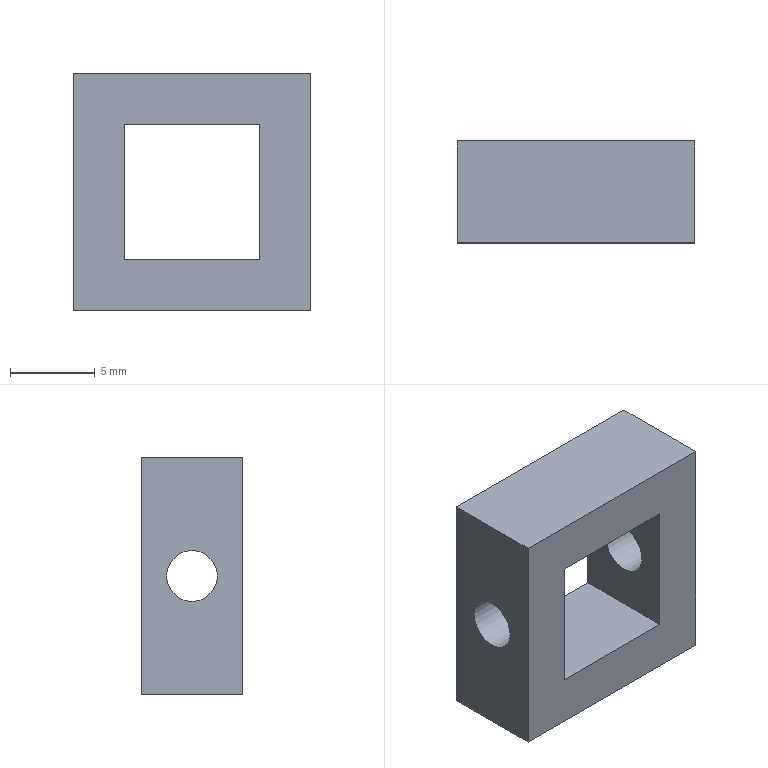Component | NX | PISTON_BLOCK_ASSEMBLY | 1 solid | 12 faces | box 14 x 6 x 14 mm | volume 750 mm3 | plane 10 | cylinder 2 | commonest cylinder face diameters 3 x2
STEP:
#1=CARTESIAN_POINT('',(0.,0.,0.));
#2=DIRECTION('',(0.,0.,1.));
#3=DIRECTION('',(1.,0.,0.));
#4=AXIS2_PLACEMENT_3D('',#1,#2,#3);
#5=CARTESIAN_POINT('',(-96.724,-9.25,41.));
#6=VERTEX_POINT('',#5);
#7=CARTESIAN_POINT('',(-96.724,-10.75,41.));
#8=DIRECTION('',(-1.,0.,0.));
#9=DIRECTION('',(0.,1.,0.));
#10=AXIS2_PLACEMENT_3D('',#7,#8,#9);
#11=CIRCLE('',#10,1.5);
#12=CARTESIAN_POINT('',(-96.724,-7.75,45.));
#13=DIRECTION('',(-1.,0.,0.));
#14=DIRECTION('',(0.,1.,0.));
#15=AXIS2_PLACEMENT_3D('',#12,#13,#14);
#16=PLANE('',#15);
#17=CARTESIAN_POINT('',(-3.,4.));
#18=DIRECTION('',(1.,0.));
#19=AXIS2_PLACEMENT_2D('',#17,#18);
#20=CIRCLE('',#19,1.5);
#21=(GEOMETRIC_REPRESENTATION_CONTEXT(2)PARAMETRIC_REPRESENTATION_CONTEXT()REPRESENTATION_CONTEXT('',''));
#22=DEFINITIONAL_REPRESENTATION('',(#20),#21);
#23=PCURVE('',#16,#22);
#24=CARTESIAN_POINT('',(-85.724,-10.75,41.));
#25=DIRECTION('',(-1.,0.,0.));
#26=DIRECTION('',(0.,1.,0.));
#27=AXIS2_PLACEMENT_3D('',#24,#25,#26);
#28=CYLINDRICAL_SURFACE('',#27,1.5);
#29=CARTESIAN_POINT('',(0.,11.));
#30=DIRECTION('',(1.,0.));
#31=VECTOR('',#30,1.);
#32=LINE('',#29,#31);
#33=(GEOMETRIC_REPRESENTATION_CONTEXT(2)PARAMETRIC_REPRESENTATION_CONTEXT()REPRESENTATION_CONTEXT('',''));
#34=DEFINITIONAL_REPRESENTATION('',(#32),#33);
#35=PCURVE('',#28,#34);
#36=SURFACE_CURVE('',#11,(#23,#35),.PCURVE_S1.);
#37=EDGE_CURVE('',#6,#6,#36,.T.);
#38=ORIENTED_EDGE('',*,*,#37,.T.);
#39=EDGE_LOOP('',(#38));
#40=FACE_BOUND('',#39,.T.);
#41=CARTESIAN_POINT('',(-96.724,-13.75,45.));
#42=VERTEX_POINT('',#41);
#43=CARTESIAN_POINT('',(-96.724,-13.75,37.));
#44=VERTEX_POINT('',#43);
#45=CARTESIAN_POINT('',(-96.724,-13.75,45.));
#46=DIRECTION('',(0.,0.,-1.));
#47=VECTOR('',#46,1.);
#48=LINE('',#45,#47);
#49=CARTESIAN_POINT('',(-6.,0.));
#50=DIRECTION('',(0.,1.));
#51=VECTOR('',#50,1.);
#52=LINE('',#49,#51);
#53=(GEOMETRIC_REPRESENTATION_CONTEXT(2)PARAMETRIC_REPRESENTATION_CONTEXT()REPRESENTATION_CONTEXT('',''));
#54=DEFINITIONAL_REPRESENTATION('',(#52),#53);
#55=PCURVE('',#16,#54);
#56=CARTESIAN_POINT('',(-92.724,-13.75,41.));
#57=DIRECTION('',(0.,-1.,0.));
#58=DIRECTION('',(-1.,0.,0.));
#59=AXIS2_PLACEMENT_3D('',#56,#57,#58);
#60=PLANE('',#59);
#61=CARTESIAN_POINT('',(4.,-4.));
#62=DIRECTION('',(0.,1.));
#63=VECTOR('',#62,1.);
#64=LINE('',#61,#63);
#65=(GEOMETRIC_REPRESENTATION_CONTEXT(2)PARAMETRIC_REPRESENTATION_CONTEXT()REPRESENTATION_CONTEXT('',''));
#66=DEFINITIONAL_REPRESENTATION('',(#64),#65);
#67=PCURVE('',#60,#66);
#68=SURFACE_CURVE('',#48,(#55,#67),.PCURVE_S1.);
#69=EDGE_CURVE('',#42,#44,#68,.T.);
#70=ORIENTED_EDGE('',*,*,#69,.T.);
#71=CARTESIAN_POINT('',(-96.724,-7.75,37.));
#72=VERTEX_POINT('',#71);
#73=CARTESIAN_POINT('',(-96.724,-7.75,37.));
#74=DIRECTION('',(0.,-1.,0.));
#75=VECTOR('',#74,1.);
#76=LINE('',#73,#75);
#77=CARTESIAN_POINT('',(0.,8.));
#78=DIRECTION('',(-1.,0.));
#79=VECTOR('',#78,1.);
#80=LINE('',#77,#79);
#81=(GEOMETRIC_REPRESENTATION_CONTEXT(2)PARAMETRIC_REPRESENTATION_CONTEXT()REPRESENTATION_CONTEXT('',''));
#82=DEFINITIONAL_REPRESENTATION('',(#80),#81);
#83=PCURVE('',#16,#82);
#84=CARTESIAN_POINT('',(-96.724,-7.75,37.));
#85=DIRECTION('',(0.,0.,-1.));
#86=DIRECTION('',(0.,1.,0.));
#87=AXIS2_PLACEMENT_3D('',#84,#85,#86);
#88=PLANE('',#87);
#89=CARTESIAN_POINT('',(0.,0.));
#90=DIRECTION('',(-1.,0.));
#91=VECTOR('',#90,1.);
#92=LINE('',#89,#91);
#93=(GEOMETRIC_REPRESENTATION_CONTEXT(2)PARAMETRIC_REPRESENTATION_CONTEXT()REPRESENTATION_CONTEXT('',''));
#94=DEFINITIONAL_REPRESENTATION('',(#92),#93);
#95=PCURVE('',#88,#94);
#96=SURFACE_CURVE('',#76,(#83,#95),.PCURVE_S1.);
#97=EDGE_CURVE('',#72,#44,#96,.T.);
#98=ORIENTED_EDGE('',*,*,#97,.F.);
#99=CARTESIAN_POINT('',(-96.724,-7.75,45.));
#100=VERTEX_POINT('',#99);
#101=CARTESIAN_POINT('',(-96.724,-7.75,45.));
#102=DIRECTION('',(0.,0.,-1.));
#103=VECTOR('',#102,1.);
#104=LINE('',#101,#103);
#105=CARTESIAN_POINT('',(0.,0.));
#106=DIRECTION('',(0.,1.));
#107=VECTOR('',#106,1.);
#108=LINE('',#105,#107);
#109=(GEOMETRIC_REPRESENTATION_CONTEXT(2)PARAMETRIC_REPRESENTATION_CONTEXT()REPRESENTATION_CONTEXT('',''));
#110=DEFINITIONAL_REPRESENTATION('',(#108),#109);
#111=PCURVE('',#16,#110);
#112=CARTESIAN_POINT('',(-92.724,-7.75,41.));
#113=DIRECTION('',(0.,-1.,0.));
#114=DIRECTION('',(-1.,0.,0.));
#115=AXIS2_PLACEMENT_3D('',#112,#113,#114);
#116=PLANE('',#115);
#117=CARTESIAN_POINT('',(4.,-4.));
#118=DIRECTION('',(0.,1.));
#119=VECTOR('',#118,1.);
#120=LINE('',#117,#119);
#121=(GEOMETRIC_REPRESENTATION_CONTEXT(2)PARAMETRIC_REPRESENTATION_CONTEXT()REPRESENTATION_CONTEXT('',''));
#122=DEFINITIONAL_REPRESENTATION('',(#120),#121);
#123=PCURVE('',#116,#122);
#124=SURFACE_CURVE('',#104,(#111,#123),.PCURVE_S1.);
#125=EDGE_CURVE('',#100,#72,#124,.T.);
#126=ORIENTED_EDGE('',*,*,#125,.F.);
#127=CARTESIAN_POINT('',(-96.724,-7.75,45.));
#128=DIRECTION('',(0.,-1.,0.));
#129=VECTOR('',#128,1.);
#130=LINE('',#127,#129);
#131=CARTESIAN_POINT('',(0.,0.));
#132=DIRECTION('',(-1.,0.));
#133=VECTOR('',#132,1.);
#134=LINE('',#131,#133);
#135=(GEOMETRIC_REPRESENTATION_CONTEXT(2)PARAMETRIC_REPRESENTATION_CONTEXT()REPRESENTATION_CONTEXT('',''));
#136=DEFINITIONAL_REPRESENTATION('',(#134),#135);
#137=PCURVE('',#16,#136);
#138=CARTESIAN_POINT('',(-88.724,-7.75,45.));
#139=DIRECTION('',(0.,0.,1.));
#140=DIRECTION('',(0.,-1.,0.));
#141=AXIS2_PLACEMENT_3D('',#138,#139,#140);
#142=PLANE('',#141);
#143=CARTESIAN_POINT('',(0.,-8.));
#144=DIRECTION('',(1.,0.));
#145=VECTOR('',#144,1.);
#146=LINE('',#143,#145);
#147=(GEOMETRIC_REPRESENTATION_CONTEXT(2)PARAMETRIC_REPRESENTATION_CONTEXT()REPRESENTATION_CONTEXT('',''));
#148=DEFINITIONAL_REPRESENTATION('',(#146),#147);
#149=PCURVE('',#142,#148);
#150=SURFACE_CURVE('',#130,(#137,#149),.PCURVE_S1.);
#151=EDGE_CURVE('',#100,#42,#150,.T.);
#152=ORIENTED_EDGE('',*,*,#151,.T.);
#153=EDGE_LOOP('',(#70,#98,#126,#152));
#154=FACE_BOUND('',#153,.T.);
#155=ADVANCED_FACE('',(#40,#154),#16,.F.);
#156=CARTESIAN_POINT('',(-88.724,-13.75,45.));
#157=VERTEX_POINT('',#156);
#158=CARTESIAN_POINT('',(-88.724,-13.75,45.));
#159=DIRECTION('',(-1.,0.,0.));
#160=VECTOR('',#159,1.);
#161=LINE('',#158,#160);
#162=CARTESIAN_POINT('',(6.,0.));
#163=DIRECTION('',(0.,-1.));
#164=VECTOR('',#163,1.);
#165=LINE('',#162,#164);
#166=(GEOMETRIC_REPRESENTATION_CONTEXT(2)PARAMETRIC_REPRESENTATION_CONTEXT()REPRESENTATION_CONTEXT('',''));
#167=DEFINITIONAL_REPRESENTATION('',(#165),#166);
#168=PCURVE('',#142,#167);
#169=CARTESIAN_POINT('',(-4.,-4.));
#170=DIRECTION('',(1.,0.));
#171=VECTOR('',#170,1.);
#172=LINE('',#169,#171);
#173=(GEOMETRIC_REPRESENTATION_CONTEXT(2)PARAMETRIC_REPRESENTATION_CONTEXT()REPRESENTATION_CONTEXT('',''));
#174=DEFINITIONAL_REPRESENTATION('',(#172),#173);
#175=PCURVE('',#60,#174);
#176=SURFACE_CURVE('',#161,(#168,#175),.PCURVE_S1.);
#177=EDGE_CURVE('',#157,#42,#176,.T.);
#178=ORIENTED_EDGE('',*,*,#177,.T.);
#179=ORIENTED_EDGE('',*,*,#151,.F.);
#180=CARTESIAN_POINT('',(-88.724,-7.75,45.));
#181=VERTEX_POINT('',#180);
#182=CARTESIAN_POINT('',(-88.724,-7.75,45.));
#183=DIRECTION('',(-1.,0.,0.));
#184=VECTOR('',#183,1.);
#185=LINE('',#182,#184);
#186=CARTESIAN_POINT('',(0.,0.));
#187=DIRECTION('',(0.,-1.));
#188=VECTOR('',#187,1.);
#189=LINE('',#186,#188);
#190=(GEOMETRIC_REPRESENTATION_CONTEXT(2)PARAMETRIC_REPRESENTATION_CONTEXT()REPRESENTATION_CONTEXT('',''));
#191=DEFINITIONAL_REPRESENTATION('',(#189),#190);
#192=PCURVE('',#142,#191);
#193=CARTESIAN_POINT('',(-4.,-4.));
#194=DIRECTION('',(1.,0.));
#195=VECTOR('',#194,1.);
#196=LINE('',#193,#195);
#197=(GEOMETRIC_REPRESENTATION_CONTEXT(2)PARAMETRIC_REPRESENTATION_CONTEXT()REPRESENTATION_CONTEXT('',''));
#198=DEFINITIONAL_REPRESENTATION('',(#196),#197);
#199=PCURVE('',#116,#198);
#200=SURFACE_CURVE('',#185,(#192,#199),.PCURVE_S1.);
#201=EDGE_CURVE('',#181,#100,#200,.T.);
#202=ORIENTED_EDGE('',*,*,#201,.F.);
#203=CARTESIAN_POINT('',(-88.724,-7.75,45.));
#204=DIRECTION('',(0.,-1.,0.));
#205=VECTOR('',#204,1.);
#206=LINE('',#203,#205);
#207=CARTESIAN_POINT('',(0.,0.));
#208=DIRECTION('',(1.,0.));
#209=VECTOR('',#208,1.);
#210=LINE('',#207,#209);
#211=(GEOMETRIC_REPRESENTATION_CONTEXT(2)PARAMETRIC_REPRESENTATION_CONTEXT()REPRESENTATION_CONTEXT('',''));
#212=DEFINITIONAL_REPRESENTATION('',(#210),#211);
#213=PCURVE('',#142,#212);
#214=CARTESIAN_POINT('',(-88.724,-7.75,37.));
#215=DIRECTION('',(1.,0.,0.));
#216=DIRECTION('',(0.,-1.,0.));
#217=AXIS2_PLACEMENT_3D('',#214,#215,#216);
#218=PLANE('',#217);
#219=CARTESIAN_POINT('',(0.,-8.));
#220=DIRECTION('',(1.,0.));
#221=VECTOR('',#220,1.);
#222=LINE('',#219,#221);
#223=(GEOMETRIC_REPRESENTATION_CONTEXT(2)PARAMETRIC_REPRESENTATION_CONTEXT()REPRESENTATION_CONTEXT('',''));
#224=DEFINITIONAL_REPRESENTATION('',(#222),#223);
#225=PCURVE('',#218,#224);
#226=SURFACE_CURVE('',#206,(#213,#225),.PCURVE_S1.);
#227=EDGE_CURVE('',#181,#157,#226,.T.);
#228=ORIENTED_EDGE('',*,*,#227,.T.);
#229=EDGE_LOOP('',(#178,#179,#202,#228));
#230=FACE_BOUND('',#229,.T.);
#231=ADVANCED_FACE('',(#230),#142,.F.);
#232=CARTESIAN_POINT('',(-88.724,-12.25,41.));
#233=VERTEX_POINT('',#232);
#234=CARTESIAN_POINT('',(-88.724,-9.25,41.));
#235=VERTEX_POINT('',#234);
#236=CARTESIAN_POINT('',(-88.724,-10.75,41.));
#237=DIRECTION('',(1.,0.,0.));
#238=DIRECTION('',(0.,-1.,0.));
#239=AXIS2_PLACEMENT_3D('',#236,#237,#238);
#240=CIRCLE('',#239,1.5);
#241=CARTESIAN_POINT('',(3.,-4.));
#242=DIRECTION('',(1.,0.));
#243=AXIS2_PLACEMENT_2D('',#241,#242);
#244=CIRCLE('',#243,1.5);
#245=(GEOMETRIC_REPRESENTATION_CONTEXT(2)PARAMETRIC_REPRESENTATION_CONTEXT()REPRESENTATION_CONTEXT('',''));
#246=DEFINITIONAL_REPRESENTATION('',(#244),#245);
#247=PCURVE('',#218,#246);
#248=CARTESIAN_POINT('',(-85.724,-10.75,41.));
#249=DIRECTION('',(-1.,0.,0.));
#250=DIRECTION('',(0.,1.,0.));
#251=AXIS2_PLACEMENT_3D('',#248,#249,#250);
#252=CYLINDRICAL_SURFACE('',#251,1.5);
#253=CARTESIAN_POINT('',(3.142,3.));
#254=DIRECTION('',(-1.,0.));
#255=VECTOR('',#254,1.);
#256=LINE('',#253,#255);
#257=(GEOMETRIC_REPRESENTATION_CONTEXT(2)PARAMETRIC_REPRESENTATION_CONTEXT()REPRESENTATION_CONTEXT('',''));
#258=DEFINITIONAL_REPRESENTATION('',(#256),#257);
#259=PCURVE('',#252,#258);
#260=SURFACE_CURVE('',#240,(#247,#259),.PCURVE_S1.);
#261=EDGE_CURVE('',#233,#235,#260,.T.);
#262=ORIENTED_EDGE('',*,*,#261,.T.);
#263=CARTESIAN_POINT('',(-88.724,-10.75,41.));
#264=DIRECTION('',(1.,0.,0.));
#265=DIRECTION('',(0.,-1.,0.));
#266=AXIS2_PLACEMENT_3D('',#263,#264,#265);
#267=CIRCLE('',#266,1.5);
#268=CARTESIAN_POINT('',(3.,-4.));
#269=DIRECTION('',(1.,0.));
#270=AXIS2_PLACEMENT_2D('',#268,#269);
#271=CIRCLE('',#270,1.5);
#272=(GEOMETRIC_REPRESENTATION_CONTEXT(2)PARAMETRIC_REPRESENTATION_CONTEXT()REPRESENTATION_CONTEXT('',''));
#273=DEFINITIONAL_REPRESENTATION('',(#271),#272);
#274=PCURVE('',#218,#273);
#275=CARTESIAN_POINT('',(9.425,3.));
#276=DIRECTION('',(-1.,0.));
#277=VECTOR('',#276,1.);
#278=LINE('',#275,#277);
#279=(GEOMETRIC_REPRESENTATION_CONTEXT(2)PARAMETRIC_REPRESENTATION_CONTEXT()REPRESENTATION_CONTEXT('',''));
#280=DEFINITIONAL_REPRESENTATION('',(#278),#279);
#281=PCURVE('',#252,#280);
#282=SURFACE_CURVE('',#267,(#274,#281),.PCURVE_S1.);
#283=EDGE_CURVE('',#235,#233,#282,.T.);
#284=ORIENTED_EDGE('',*,*,#283,.T.);
#285=EDGE_LOOP('',(#262,#284));
#286=FACE_BOUND('',#285,.T.);
#287=CARTESIAN_POINT('',(-88.724,-13.75,37.));
#288=VERTEX_POINT('',#287);
#289=CARTESIAN_POINT('',(-88.724,-13.75,37.));
#290=DIRECTION('',(0.,0.,1.));
#291=VECTOR('',#290,1.);
#292=LINE('',#289,#291);
#293=CARTESIAN_POINT('',(6.,0.));
#294=DIRECTION('',(0.,-1.));
#295=VECTOR('',#294,1.);
#296=LINE('',#293,#295);
#297=(GEOMETRIC_REPRESENTATION_CONTEXT(2)PARAMETRIC_REPRESENTATION_CONTEXT()REPRESENTATION_CONTEXT('',''));
#298=DEFINITIONAL_REPRESENTATION('',(#296),#297);
#299=PCURVE('',#218,#298);
#300=CARTESIAN_POINT('',(-4.,4.));
#301=DIRECTION('',(0.,-1.));
#302=VECTOR('',#301,1.);
#303=LINE('',#300,#302);
#304=(GEOMETRIC_REPRESENTATION_CONTEXT(2)PARAMETRIC_REPRESENTATION_CONTEXT()REPRESENTATION_CONTEXT('',''));
#305=DEFINITIONAL_REPRESENTATION('',(#303),#304);
#306=PCURVE('',#60,#305);
#307=SURFACE_CURVE('',#292,(#299,#306),.PCURVE_S1.);
#308=EDGE_CURVE('',#288,#157,#307,.T.);
#309=ORIENTED_EDGE('',*,*,#308,.T.);
#310=ORIENTED_EDGE('',*,*,#227,.F.);
#311=CARTESIAN_POINT('',(-88.724,-7.75,37.));
#312=VERTEX_POINT('',#311);
#313=CARTESIAN_POINT('',(-88.724,-7.75,37.));
#314=DIRECTION('',(0.,0.,1.));
#315=VECTOR('',#314,1.);
#316=LINE('',#313,#315);
#317=CARTESIAN_POINT('',(0.,0.));
#318=DIRECTION('',(0.,-1.));
#319=VECTOR('',#318,1.);
#320=LINE('',#317,#319);
#321=(GEOMETRIC_REPRESENTATION_CONTEXT(2)PARAMETRIC_REPRESENTATION_CONTEXT()REPRESENTATION_CONTEXT('',''));
#322=DEFINITIONAL_REPRESENTATION('',(#320),#321);
#323=PCURVE('',#218,#322);
#324=CARTESIAN_POINT('',(-4.,4.));
#325=DIRECTION('',(0.,-1.));
#326=VECTOR('',#325,1.);
#327=LINE('',#324,#326);
#328=(GEOMETRIC_REPRESENTATION_CONTEXT(2)PARAMETRIC_REPRESENTATION_CONTEXT()REPRESENTATION_CONTEXT('',''));
#329=DEFINITIONAL_REPRESENTATION('',(#327),#328);
#330=PCURVE('',#116,#329);
#331=SURFACE_CURVE('',#316,(#323,#330),.PCURVE_S1.);
#332=EDGE_CURVE('',#312,#181,#331,.T.);
#333=ORIENTED_EDGE('',*,*,#332,.F.);
#334=CARTESIAN_POINT('',(-88.724,-7.75,37.));
#335=DIRECTION('',(0.,-1.,0.));
#336=VECTOR('',#335,1.);
#337=LINE('',#334,#336);
#338=CARTESIAN_POINT('',(0.,0.));
#339=DIRECTION('',(1.,0.));
#340=VECTOR('',#339,1.);
#341=LINE('',#338,#340);
#342=(GEOMETRIC_REPRESENTATION_CONTEXT(2)PARAMETRIC_REPRESENTATION_CONTEXT()REPRESENTATION_CONTEXT('',''));
#343=DEFINITIONAL_REPRESENTATION('',(#341),#342);
#344=PCURVE('',#218,#343);
#345=CARTESIAN_POINT('',(0.,8.));
#346=DIRECTION('',(-1.,0.));
#347=VECTOR('',#346,1.);
#348=LINE('',#345,#347);
#349=(GEOMETRIC_REPRESENTATION_CONTEXT(2)PARAMETRIC_REPRESENTATION_CONTEXT()REPRESENTATION_CONTEXT('',''));
#350=DEFINITIONAL_REPRESENTATION('',(#348),#349);
#351=PCURVE('',#88,#350);
#352=SURFACE_CURVE('',#337,(#344,#351),.PCURVE_S1.);
#353=EDGE_CURVE('',#312,#288,#352,.T.);
#354=ORIENTED_EDGE('',*,*,#353,.T.);
#355=EDGE_LOOP('',(#309,#310,#333,#354));
#356=FACE_BOUND('',#355,.T.);
#357=ADVANCED_FACE('',(#286,#356),#218,.F.);
#358=CARTESIAN_POINT('',(-85.724,-13.75,48.));
#359=VERTEX_POINT('',#358);
#360=CARTESIAN_POINT('',(-99.724,-13.75,48.));
#361=VERTEX_POINT('',#360);
#362=CARTESIAN_POINT('',(-85.724,-13.75,48.));
#363=DIRECTION('',(-1.,0.,0.));
#364=VECTOR('',#363,1.);
#365=LINE('',#362,#364);
#366=CARTESIAN_POINT('',(-85.724,-7.75,48.));
#367=DIRECTION('',(0.,0.,1.));
#368=DIRECTION('',(0.,-1.,0.));
#369=AXIS2_PLACEMENT_3D('',#366,#367,#368);
#370=PLANE('',#369);
#371=CARTESIAN_POINT('',(6.,0.));
#372=DIRECTION('',(0.,-1.));
#373=VECTOR('',#372,1.);
#374=LINE('',#371,#373);
#375=(GEOMETRIC_REPRESENTATION_CONTEXT(2)PARAMETRIC_REPRESENTATION_CONTEXT()REPRESENTATION_CONTEXT('',''));
#376=DEFINITIONAL_REPRESENTATION('',(#374),#375);
#377=PCURVE('',#370,#376);
#378=CARTESIAN_POINT('',(-7.,-7.));
#379=DIRECTION('',(1.,0.));
#380=VECTOR('',#379,1.);
#381=LINE('',#378,#380);
#382=(GEOMETRIC_REPRESENTATION_CONTEXT(2)PARAMETRIC_REPRESENTATION_CONTEXT()REPRESENTATION_CONTEXT('',''));
#383=DEFINITIONAL_REPRESENTATION('',(#381),#382);
#384=PCURVE('',#60,#383);
#385=SURFACE_CURVE('',#365,(#377,#384),.PCURVE_S1.);
#386=EDGE_CURVE('',#359,#361,#385,.T.);
#387=ORIENTED_EDGE('',*,*,#386,.F.);
#388=CARTESIAN_POINT('',(-85.724,-7.75,48.));
#389=VERTEX_POINT('',#388);
#390=CARTESIAN_POINT('',(-85.724,-7.75,48.));
#391=DIRECTION('',(0.,-1.,0.));
#392=VECTOR('',#391,1.);
#393=LINE('',#390,#392);
#394=CARTESIAN_POINT('',(0.,0.));
#395=DIRECTION('',(1.,0.));
#396=VECTOR('',#395,1.);
#397=LINE('',#394,#396);
#398=(GEOMETRIC_REPRESENTATION_CONTEXT(2)PARAMETRIC_REPRESENTATION_CONTEXT()REPRESENTATION_CONTEXT('',''));
#399=DEFINITIONAL_REPRESENTATION('',(#397),#398);
#400=PCURVE('',#370,#399);
#401=CARTESIAN_POINT('',(-85.724,-7.75,34.));
#402=DIRECTION('',(1.,0.,0.));
#403=DIRECTION('',(0.,-1.,0.));
#404=AXIS2_PLACEMENT_3D('',#401,#402,#403);
#405=PLANE('',#404);
#406=CARTESIAN_POINT('',(0.,-14.));
#407=DIRECTION('',(1.,0.));
#408=VECTOR('',#407,1.);
#409=LINE('',#406,#408);
#410=(GEOMETRIC_REPRESENTATION_CONTEXT(2)PARAMETRIC_REPRESENTATION_CONTEXT()REPRESENTATION_CONTEXT('',''));
#411=DEFINITIONAL_REPRESENTATION('',(#409),#410);
#412=PCURVE('',#405,#411);
#413=SURFACE_CURVE('',#393,(#400,#412),.PCURVE_S1.);
#414=EDGE_CURVE('',#389,#359,#413,.T.);
#415=ORIENTED_EDGE('',*,*,#414,.F.);
#416=CARTESIAN_POINT('',(-99.724,-7.75,48.));
#417=VERTEX_POINT('',#416);
#418=CARTESIAN_POINT('',(-85.724,-7.75,48.));
#419=DIRECTION('',(-1.,0.,0.));
#420=VECTOR('',#419,1.);
#421=LINE('',#418,#420);
#422=CARTESIAN_POINT('',(0.,0.));
#423=DIRECTION('',(0.,-1.));
#424=VECTOR('',#423,1.);
#425=LINE('',#422,#424);
#426=(GEOMETRIC_REPRESENTATION_CONTEXT(2)PARAMETRIC_REPRESENTATION_CONTEXT()REPRESENTATION_CONTEXT('',''));
#427=DEFINITIONAL_REPRESENTATION('',(#425),#426);
#428=PCURVE('',#370,#427);
#429=CARTESIAN_POINT('',(-7.,-7.));
#430=DIRECTION('',(1.,0.));
#431=VECTOR('',#430,1.);
#432=LINE('',#429,#431);
#433=(GEOMETRIC_REPRESENTATION_CONTEXT(2)PARAMETRIC_REPRESENTATION_CONTEXT()REPRESENTATION_CONTEXT('',''));
#434=DEFINITIONAL_REPRESENTATION('',(#432),#433);
#435=PCURVE('',#116,#434);
#436=SURFACE_CURVE('',#421,(#428,#435),.PCURVE_S1.);
#437=EDGE_CURVE('',#389,#417,#436,.T.);
#438=ORIENTED_EDGE('',*,*,#437,.T.);
#439=CARTESIAN_POINT('',(-99.724,-7.75,48.));
#440=DIRECTION('',(0.,-1.,0.));
#441=VECTOR('',#440,1.);
#442=LINE('',#439,#441);
#443=CARTESIAN_POINT('',(0.,-14.));
#444=DIRECTION('',(1.,0.));
#445=VECTOR('',#444,1.);
#446=LINE('',#443,#445);
#447=(GEOMETRIC_REPRESENTATION_CONTEXT(2)PARAMETRIC_REPRESENTATION_CONTEXT()REPRESENTATION_CONTEXT('',''));
#448=DEFINITIONAL_REPRESENTATION('',(#446),#447);
#449=PCURVE('',#370,#448);
#450=CARTESIAN_POINT('',(-99.724,-7.75,48.));
#451=DIRECTION('',(-1.,0.,0.));
#452=DIRECTION('',(0.,1.,0.));
#453=AXIS2_PLACEMENT_3D('',#450,#451,#452);
#454=PLANE('',#453);
#455=CARTESIAN_POINT('',(0.,0.));
#456=DIRECTION('',(-1.,0.));
#457=VECTOR('',#456,1.);
#458=LINE('',#455,#457);
#459=(GEOMETRIC_REPRESENTATION_CONTEXT(2)PARAMETRIC_REPRESENTATION_CONTEXT()REPRESENTATION_CONTEXT('',''));
#460=DEFINITIONAL_REPRESENTATION('',(#458),#459);
#461=PCURVE('',#454,#460);
#462=SURFACE_CURVE('',#442,(#449,#461),.PCURVE_S1.);
#463=EDGE_CURVE('',#417,#361,#462,.T.);
#464=ORIENTED_EDGE('',*,*,#463,.T.);
#465=EDGE_LOOP('',(#387,#415,#438,#464));
#466=FACE_BOUND('',#465,.T.);
#467=ADVANCED_FACE('',(#466),#370,.T.);
#468=CARTESIAN_POINT('',(-99.724,-9.25,41.));
#469=VERTEX_POINT('',#468);
#470=CARTESIAN_POINT('',(-99.724,-10.75,41.));
#471=DIRECTION('',(-1.,0.,0.));
#472=DIRECTION('',(0.,1.,0.));
#473=AXIS2_PLACEMENT_3D('',#470,#471,#472);
#474=CIRCLE('',#473,1.5);
#475=CARTESIAN_POINT('',(-3.,7.));
#476=DIRECTION('',(1.,0.));
#477=AXIS2_PLACEMENT_2D('',#475,#476);
#478=CIRCLE('',#477,1.5);
#479=(GEOMETRIC_REPRESENTATION_CONTEXT(2)PARAMETRIC_REPRESENTATION_CONTEXT()REPRESENTATION_CONTEXT('',''));
#480=DEFINITIONAL_REPRESENTATION('',(#478),#479);
#481=PCURVE('',#454,#480);
#482=CARTESIAN_POINT('',(0.,14.));
#483=DIRECTION('',(1.,0.));
#484=VECTOR('',#483,1.);
#485=LINE('',#482,#484);
#486=(GEOMETRIC_REPRESENTATION_CONTEXT(2)PARAMETRIC_REPRESENTATION_CONTEXT()REPRESENTATION_CONTEXT('',''));
#487=DEFINITIONAL_REPRESENTATION('',(#485),#486);
#488=PCURVE('',#28,#487);
#489=SURFACE_CURVE('',#474,(#481,#488),.PCURVE_S1.);
#490=EDGE_CURVE('',#469,#469,#489,.T.);
#491=ORIENTED_EDGE('',*,*,#490,.F.);
#492=EDGE_LOOP('',(#491));
#493=FACE_BOUND('',#492,.T.);
#494=CARTESIAN_POINT('',(-99.724,-13.75,34.));
#495=VERTEX_POINT('',#494);
#496=CARTESIAN_POINT('',(-99.724,-13.75,48.));
#497=DIRECTION('',(0.,0.,-1.));
#498=VECTOR('',#497,1.);
#499=LINE('',#496,#498);
#500=CARTESIAN_POINT('',(-6.,0.));
#501=DIRECTION('',(0.,1.));
#502=VECTOR('',#501,1.);
#503=LINE('',#500,#502);
#504=(GEOMETRIC_REPRESENTATION_CONTEXT(2)PARAMETRIC_REPRESENTATION_CONTEXT()REPRESENTATION_CONTEXT('',''));
#505=DEFINITIONAL_REPRESENTATION('',(#503),#504);
#506=PCURVE('',#454,#505);
#507=CARTESIAN_POINT('',(7.,-7.));
#508=DIRECTION('',(0.,1.));
#509=VECTOR('',#508,1.);
#510=LINE('',#507,#509);
#511=(GEOMETRIC_REPRESENTATION_CONTEXT(2)PARAMETRIC_REPRESENTATION_CONTEXT()REPRESENTATION_CONTEXT('',''));
#512=DEFINITIONAL_REPRESENTATION('',(#510),#511);
#513=PCURVE('',#60,#512);
#514=SURFACE_CURVE('',#499,(#506,#513),.PCURVE_S1.);
#515=EDGE_CURVE('',#361,#495,#514,.T.);
#516=ORIENTED_EDGE('',*,*,#515,.F.);
#517=ORIENTED_EDGE('',*,*,#463,.F.);
#518=CARTESIAN_POINT('',(-99.724,-7.75,34.));
#519=VERTEX_POINT('',#518);
#520=CARTESIAN_POINT('',(-99.724,-7.75,48.));
#521=DIRECTION('',(0.,0.,-1.));
#522=VECTOR('',#521,1.);
#523=LINE('',#520,#522);
#524=CARTESIAN_POINT('',(0.,0.));
#525=DIRECTION('',(0.,1.));
#526=VECTOR('',#525,1.);
#527=LINE('',#524,#526);
#528=(GEOMETRIC_REPRESENTATION_CONTEXT(2)PARAMETRIC_REPRESENTATION_CONTEXT()REPRESENTATION_CONTEXT('',''));
#529=DEFINITIONAL_REPRESENTATION('',(#527),#528);
#530=PCURVE('',#454,#529);
#531=CARTESIAN_POINT('',(7.,-7.));
#532=DIRECTION('',(0.,1.));
#533=VECTOR('',#532,1.);
#534=LINE('',#531,#533);
#535=(GEOMETRIC_REPRESENTATION_CONTEXT(2)PARAMETRIC_REPRESENTATION_CONTEXT()REPRESENTATION_CONTEXT('',''));
#536=DEFINITIONAL_REPRESENTATION('',(#534),#535);
#537=PCURVE('',#116,#536);
#538=SURFACE_CURVE('',#523,(#530,#537),.PCURVE_S1.);
#539=EDGE_CURVE('',#417,#519,#538,.T.);
#540=ORIENTED_EDGE('',*,*,#539,.T.);
#541=CARTESIAN_POINT('',(-99.724,-7.75,34.));
#542=DIRECTION('',(0.,-1.,0.));
#543=VECTOR('',#542,1.);
#544=LINE('',#541,#543);
#545=CARTESIAN_POINT('',(0.,14.));
#546=DIRECTION('',(-1.,0.));
#547=VECTOR('',#546,1.);
#548=LINE('',#545,#547);
#549=(GEOMETRIC_REPRESENTATION_CONTEXT(2)PARAMETRIC_REPRESENTATION_CONTEXT()REPRESENTATION_CONTEXT('',''));
#550=DEFINITIONAL_REPRESENTATION('',(#548),#549);
#551=PCURVE('',#454,#550);
#552=CARTESIAN_POINT('',(-99.724,-7.75,34.));
#553=DIRECTION('',(0.,0.,-1.));
#554=DIRECTION('',(0.,1.,0.));
#555=AXIS2_PLACEMENT_3D('',#552,#553,#554);
#556=PLANE('',#555);
#557=CARTESIAN_POINT('',(0.,0.));
#558=DIRECTION('',(-1.,0.));
#559=VECTOR('',#558,1.);
#560=LINE('',#557,#559);
#561=(GEOMETRIC_REPRESENTATION_CONTEXT(2)PARAMETRIC_REPRESENTATION_CONTEXT()REPRESENTATION_CONTEXT('',''));
#562=DEFINITIONAL_REPRESENTATION('',(#560),#561);
#563=PCURVE('',#556,#562);
#564=SURFACE_CURVE('',#544,(#551,#563),.PCURVE_S1.);
#565=EDGE_CURVE('',#519,#495,#564,.T.);
#566=ORIENTED_EDGE('',*,*,#565,.T.);
#567=EDGE_LOOP('',(#516,#517,#540,#566));
#568=FACE_BOUND('',#567,.T.);
#569=ADVANCED_FACE('',(#493,#568),#454,.T.);
#570=CARTESIAN_POINT('',(-85.724,-13.75,34.));
#571=VERTEX_POINT('',#570);
#572=CARTESIAN_POINT('',(-99.724,-13.75,34.));
#573=DIRECTION('',(1.,0.,0.));
#574=VECTOR('',#573,1.);
#575=LINE('',#572,#574);
#576=CARTESIAN_POINT('',(-6.,0.));
#577=DIRECTION('',(0.,1.));
#578=VECTOR('',#577,1.);
#579=LINE('',#576,#578);
#580=(GEOMETRIC_REPRESENTATION_CONTEXT(2)PARAMETRIC_REPRESENTATION_CONTEXT()REPRESENTATION_CONTEXT('',''));
#581=DEFINITIONAL_REPRESENTATION('',(#579),#580);
#582=PCURVE('',#556,#581);
#583=CARTESIAN_POINT('',(7.,7.));
#584=DIRECTION('',(-1.,0.));
#585=VECTOR('',#584,1.);
#586=LINE('',#583,#585);
#587=(GEOMETRIC_REPRESENTATION_CONTEXT(2)PARAMETRIC_REPRESENTATION_CONTEXT()REPRESENTATION_CONTEXT('',''));
#588=DEFINITIONAL_REPRESENTATION('',(#586),#587);
#589=PCURVE('',#60,#588);
#590=SURFACE_CURVE('',#575,(#582,#589),.PCURVE_S1.);
#591=EDGE_CURVE('',#495,#571,#590,.T.);
#592=ORIENTED_EDGE('',*,*,#591,.F.);
#593=ORIENTED_EDGE('',*,*,#565,.F.);
#594=CARTESIAN_POINT('',(-85.724,-7.75,34.));
#595=VERTEX_POINT('',#594);
#596=CARTESIAN_POINT('',(-99.724,-7.75,34.));
#597=DIRECTION('',(1.,0.,0.));
#598=VECTOR('',#597,1.);
#599=LINE('',#596,#598);
#600=CARTESIAN_POINT('',(0.,0.));
#601=DIRECTION('',(0.,1.));
#602=VECTOR('',#601,1.);
#603=LINE('',#600,#602);
#604=(GEOMETRIC_REPRESENTATION_CONTEXT(2)PARAMETRIC_REPRESENTATION_CONTEXT()REPRESENTATION_CONTEXT('',''));
#605=DEFINITIONAL_REPRESENTATION('',(#603),#604);
#606=PCURVE('',#556,#605);
#607=CARTESIAN_POINT('',(7.,7.));
#608=DIRECTION('',(-1.,0.));
#609=VECTOR('',#608,1.);
#610=LINE('',#607,#609);
#611=(GEOMETRIC_REPRESENTATION_CONTEXT(2)PARAMETRIC_REPRESENTATION_CONTEXT()REPRESENTATION_CONTEXT('',''));
#612=DEFINITIONAL_REPRESENTATION('',(#610),#611);
#613=PCURVE('',#116,#612);
#614=SURFACE_CURVE('',#599,(#606,#613),.PCURVE_S1.);
#615=EDGE_CURVE('',#519,#595,#614,.T.);
#616=ORIENTED_EDGE('',*,*,#615,.T.);
#617=CARTESIAN_POINT('',(-85.724,-7.75,34.));
#618=DIRECTION('',(0.,-1.,0.));
#619=VECTOR('',#618,1.);
#620=LINE('',#617,#619);
#621=CARTESIAN_POINT('',(0.,14.));
#622=DIRECTION('',(-1.,0.));
#623=VECTOR('',#622,1.);
#624=LINE('',#621,#623);
#625=(GEOMETRIC_REPRESENTATION_CONTEXT(2)PARAMETRIC_REPRESENTATION_CONTEXT()REPRESENTATION_CONTEXT('',''));
#626=DEFINITIONAL_REPRESENTATION('',(#624),#625);
#627=PCURVE('',#556,#626);
#628=CARTESIAN_POINT('',(0.,0.));
#629=DIRECTION('',(1.,0.));
#630=VECTOR('',#629,1.);
#631=LINE('',#628,#630);
#632=(GEOMETRIC_REPRESENTATION_CONTEXT(2)PARAMETRIC_REPRESENTATION_CONTEXT()REPRESENTATION_CONTEXT('',''));
#633=DEFINITIONAL_REPRESENTATION('',(#631),#632);
#634=PCURVE('',#405,#633);
#635=SURFACE_CURVE('',#620,(#627,#634),.PCURVE_S1.);
#636=EDGE_CURVE('',#595,#571,#635,.T.);
#637=ORIENTED_EDGE('',*,*,#636,.T.);
#638=EDGE_LOOP('',(#592,#593,#616,#637));
#639=FACE_BOUND('',#638,.T.);
#640=ADVANCED_FACE('',(#639),#556,.T.);
#641=CARTESIAN_POINT('',(-85.724,-9.25,41.));
#642=VERTEX_POINT('',#641);
#643=CARTESIAN_POINT('',(-85.724,-10.75,41.));
#644=DIRECTION('',(-1.,0.,0.));
#645=DIRECTION('',(0.,1.,0.));
#646=AXIS2_PLACEMENT_3D('',#643,#644,#645);
#647=CIRCLE('',#646,1.5);
#648=CARTESIAN_POINT('',(1.5,-7.));
#649=CARTESIAN_POINT('',(1.5,-4.402));
#650=CARTESIAN_POINT('',(3.75,-5.701));
#651=CARTESIAN_POINT('',(6.,-7.));
#652=CARTESIAN_POINT('',(3.75,-8.299));
#653=CARTESIAN_POINT('',(1.5,-9.598));
#654=CARTESIAN_POINT('',(1.5,-7.));
#655=(BOUNDED_CURVE()B_SPLINE_CURVE(2,(#648,#649,#650,#651,#652,#653,#654),.UNSPECIFIED.,.T.,.F.)B_SPLINE_CURVE_WITH_KNOTS((1,2,2,2,2,1),(-2.094,0.,2.094,4.189,6.283,8.378),.UNSPECIFIED.)CURVE()GEOMETRIC_REPRESENTATION_ITEM()RATIONAL_B_SPLINE_CURVE((1.,0.5,1.,0.5,1.,0.5,1.))REPRESENTATION_ITEM(''));
#656=(GEOMETRIC_REPRESENTATION_CONTEXT(2)PARAMETRIC_REPRESENTATION_CONTEXT()REPRESENTATION_CONTEXT('',''));
#657=DEFINITIONAL_REPRESENTATION('',(#655),#656);
#658=PCURVE('',#405,#657);
#659=CARTESIAN_POINT('',(0.,0.));
#660=DIRECTION('',(1.,0.));
#661=VECTOR('',#660,1.);
#662=LINE('',#659,#661);
#663=(GEOMETRIC_REPRESENTATION_CONTEXT(2)PARAMETRIC_REPRESENTATION_CONTEXT()REPRESENTATION_CONTEXT('',''));
#664=DEFINITIONAL_REPRESENTATION('',(#662),#663);
#665=PCURVE('',#252,#664);
#666=SURFACE_CURVE('',#647,(#658,#665),.PCURVE_S1.);
#667=EDGE_CURVE('',#642,#642,#666,.T.);
#668=ORIENTED_EDGE('',*,*,#667,.T.);
#669=EDGE_LOOP('',(#668));
#670=FACE_BOUND('',#669,.T.);
#671=CARTESIAN_POINT('',(-85.724,-13.75,34.));
#672=DIRECTION('',(0.,0.,1.));
#673=VECTOR('',#672,1.);
#674=LINE('',#671,#673);
#675=CARTESIAN_POINT('',(6.,0.));
#676=DIRECTION('',(0.,-1.));
#677=VECTOR('',#676,1.);
#678=LINE('',#675,#677);
#679=(GEOMETRIC_REPRESENTATION_CONTEXT(2)PARAMETRIC_REPRESENTATION_CONTEXT()REPRESENTATION_CONTEXT('',''));
#680=DEFINITIONAL_REPRESENTATION('',(#678),#679);
#681=PCURVE('',#405,#680);
#682=CARTESIAN_POINT('',(-7.,7.));
#683=DIRECTION('',(0.,-1.));
#684=VECTOR('',#683,1.);
#685=LINE('',#682,#684);
#686=(GEOMETRIC_REPRESENTATION_CONTEXT(2)PARAMETRIC_REPRESENTATION_CONTEXT()REPRESENTATION_CONTEXT('',''));
#687=DEFINITIONAL_REPRESENTATION('',(#685),#686);
#688=PCURVE('',#60,#687);
#689=SURFACE_CURVE('',#674,(#681,#688),.PCURVE_S1.);
#690=EDGE_CURVE('',#571,#359,#689,.T.);
#691=ORIENTED_EDGE('',*,*,#690,.F.);
#692=ORIENTED_EDGE('',*,*,#636,.F.);
#693=CARTESIAN_POINT('',(-85.724,-7.75,34.));
#694=DIRECTION('',(0.,0.,1.));
#695=VECTOR('',#694,1.);
#696=LINE('',#693,#695);
#697=CARTESIAN_POINT('',(0.,0.));
#698=DIRECTION('',(0.,-1.));
#699=VECTOR('',#698,1.);
#700=LINE('',#697,#699);
#701=(GEOMETRIC_REPRESENTATION_CONTEXT(2)PARAMETRIC_REPRESENTATION_CONTEXT()REPRESENTATION_CONTEXT('',''));
#702=DEFINITIONAL_REPRESENTATION('',(#700),#701);
#703=PCURVE('',#405,#702);
#704=CARTESIAN_POINT('',(-7.,7.));
#705=DIRECTION('',(0.,-1.));
#706=VECTOR('',#705,1.);
#707=LINE('',#704,#706);
#708=(GEOMETRIC_REPRESENTATION_CONTEXT(2)PARAMETRIC_REPRESENTATION_CONTEXT()REPRESENTATION_CONTEXT('',''));
#709=DEFINITIONAL_REPRESENTATION('',(#707),#708);
#710=PCURVE('',#116,#709);
#711=SURFACE_CURVE('',#696,(#703,#710),.PCURVE_S1.);
#712=EDGE_CURVE('',#595,#389,#711,.T.);
#713=ORIENTED_EDGE('',*,*,#712,.T.);
#714=ORIENTED_EDGE('',*,*,#414,.T.);
#715=EDGE_LOOP('',(#691,#692,#713,#714));
#716=FACE_BOUND('',#715,.T.);
#717=ADVANCED_FACE('',(#670,#716),#405,.T.);
#718=CARTESIAN_POINT('',(-96.724,-13.75,37.));
#719=DIRECTION('',(1.,0.,0.));
#720=VECTOR('',#719,1.);
#721=LINE('',#718,#720);
#722=CARTESIAN_POINT('',(-6.,0.));
#723=DIRECTION('',(0.,1.));
#724=VECTOR('',#723,1.);
#725=LINE('',#722,#724);
#726=(GEOMETRIC_REPRESENTATION_CONTEXT(2)PARAMETRIC_REPRESENTATION_CONTEXT()REPRESENTATION_CONTEXT('',''));
#727=DEFINITIONAL_REPRESENTATION('',(#725),#726);
#728=PCURVE('',#88,#727);
#729=CARTESIAN_POINT('',(4.,4.));
#730=DIRECTION('',(-1.,0.));
#731=VECTOR('',#730,1.);
#732=LINE('',#729,#731);
#733=(GEOMETRIC_REPRESENTATION_CONTEXT(2)PARAMETRIC_REPRESENTATION_CONTEXT()REPRESENTATION_CONTEXT('',''));
#734=DEFINITIONAL_REPRESENTATION('',(#732),#733);
#735=PCURVE('',#60,#734);
#736=SURFACE_CURVE('',#721,(#728,#735),.PCURVE_S1.);
#737=EDGE_CURVE('',#44,#288,#736,.T.);
#738=ORIENTED_EDGE('',*,*,#737,.T.);
#739=ORIENTED_EDGE('',*,*,#353,.F.);
#740=CARTESIAN_POINT('',(-96.724,-7.75,37.));
#741=DIRECTION('',(1.,0.,0.));
#742=VECTOR('',#741,1.);
#743=LINE('',#740,#742);
#744=CARTESIAN_POINT('',(0.,0.));
#745=DIRECTION('',(0.,1.));
#746=VECTOR('',#745,1.);
#747=LINE('',#744,#746);
#748=(GEOMETRIC_REPRESENTATION_CONTEXT(2)PARAMETRIC_REPRESENTATION_CONTEXT()REPRESENTATION_CONTEXT('',''));
#749=DEFINITIONAL_REPRESENTATION('',(#747),#748);
#750=PCURVE('',#88,#749);
#751=CARTESIAN_POINT('',(4.,4.));
#752=DIRECTION('',(-1.,0.));
#753=VECTOR('',#752,1.);
#754=LINE('',#751,#753);
#755=(GEOMETRIC_REPRESENTATION_CONTEXT(2)PARAMETRIC_REPRESENTATION_CONTEXT()REPRESENTATION_CONTEXT('',''));
#756=DEFINITIONAL_REPRESENTATION('',(#754),#755);
#757=PCURVE('',#116,#756);
#758=SURFACE_CURVE('',#743,(#750,#757),.PCURVE_S1.);
#759=EDGE_CURVE('',#72,#312,#758,.T.);
#760=ORIENTED_EDGE('',*,*,#759,.F.);
#761=ORIENTED_EDGE('',*,*,#97,.T.);
#762=EDGE_LOOP('',(#738,#739,#760,#761));
#763=FACE_BOUND('',#762,.T.);
#764=ADVANCED_FACE('',(#763),#88,.F.);
#765=ORIENTED_EDGE('',*,*,#437,.F.);
#766=ORIENTED_EDGE('',*,*,#712,.F.);
#767=ORIENTED_EDGE('',*,*,#615,.F.);
#768=ORIENTED_EDGE('',*,*,#539,.F.);
#769=EDGE_LOOP('',(#765,#766,#767,#768));
#770=FACE_BOUND('',#769,.T.);
#771=ORIENTED_EDGE('',*,*,#125,.T.);
#772=ORIENTED_EDGE('',*,*,#759,.T.);
#773=ORIENTED_EDGE('',*,*,#332,.T.);
#774=ORIENTED_EDGE('',*,*,#201,.T.);
#775=EDGE_LOOP('',(#771,#772,#773,#774));
#776=FACE_BOUND('',#775,.T.);
#777=ADVANCED_FACE('',(#770,#776),#116,.F.);
#778=ORIENTED_EDGE('',*,*,#386,.T.);
#779=ORIENTED_EDGE('',*,*,#515,.T.);
#780=ORIENTED_EDGE('',*,*,#591,.T.);
#781=ORIENTED_EDGE('',*,*,#690,.T.);
#782=EDGE_LOOP('',(#778,#779,#780,#781));
#783=FACE_BOUND('',#782,.T.);
#784=ORIENTED_EDGE('',*,*,#69,.F.);
#785=ORIENTED_EDGE('',*,*,#177,.F.);
#786=ORIENTED_EDGE('',*,*,#308,.F.);
#787=ORIENTED_EDGE('',*,*,#737,.F.);
#788=EDGE_LOOP('',(#784,#785,#786,#787));
#789=FACE_BOUND('',#788,.T.);
#790=ADVANCED_FACE('',(#783,#789),#60,.T.);
#791=ORIENTED_EDGE('',*,*,#667,.T.);
#792=CARTESIAN_POINT('',(-85.724,-9.25,41.));
#793=CARTESIAN_POINT('',(-88.724,-9.25,41.));
#794=B_SPLINE_CURVE_WITH_KNOTS('',1,(#792,#793),.UNSPECIFIED.,.F.,.F.,(2,2),(0.,3.),.PIECEWISE_BEZIER_KNOTS.);
#795=CARTESIAN_POINT('',(6.283,0.));
#796=DIRECTION('',(0.,1.));
#797=VECTOR('',#796,1.);
#798=LINE('',#795,#797);
#799=(GEOMETRIC_REPRESENTATION_CONTEXT(2)PARAMETRIC_REPRESENTATION_CONTEXT()REPRESENTATION_CONTEXT('',''));
#800=DEFINITIONAL_REPRESENTATION('',(#798),#799);
#801=PCURVE('',#252,#800);
#802=CARTESIAN_POINT('',(0.,0.));
#803=DIRECTION('',(0.,1.));
#804=VECTOR('',#803,1.);
#805=LINE('',#802,#804);
#806=(GEOMETRIC_REPRESENTATION_CONTEXT(2)PARAMETRIC_REPRESENTATION_CONTEXT()REPRESENTATION_CONTEXT('',''));
#807=DEFINITIONAL_REPRESENTATION('',(#805),#806);
#808=PCURVE('',#252,#807);
#809=SEAM_CURVE('',#794,(#801,#808),.PCURVE_S1.);
#810=EDGE_CURVE('',#642,#235,#809,.T.);
#811=ORIENTED_EDGE('',*,*,#810,.T.);
#812=ORIENTED_EDGE('',*,*,#283,.T.);
#813=ORIENTED_EDGE('',*,*,#261,.T.);
#814=ORIENTED_EDGE('',*,*,#810,.F.);
#815=EDGE_LOOP('',(#791,#811,#812,#813,#814));
#816=FACE_BOUND('',#815,.F.);
#817=ADVANCED_FACE('',(#816),#252,.F.);
#818=ORIENTED_EDGE('',*,*,#490,.F.);
#819=CARTESIAN_POINT('',(-96.724,-9.25,41.));
#820=CARTESIAN_POINT('',(-99.724,-9.25,41.));
#821=B_SPLINE_CURVE_WITH_KNOTS('',1,(#819,#820),.UNSPECIFIED.,.F.,.F.,(2,2),(11.,14.),.PIECEWISE_BEZIER_KNOTS.);
#822=CARTESIAN_POINT('',(0.,0.));
#823=DIRECTION('',(0.,1.));
#824=VECTOR('',#823,1.);
#825=LINE('',#822,#824);
#826=(GEOMETRIC_REPRESENTATION_CONTEXT(2)PARAMETRIC_REPRESENTATION_CONTEXT()REPRESENTATION_CONTEXT('',''));
#827=DEFINITIONAL_REPRESENTATION('',(#825),#826);
#828=PCURVE('',#28,#827);
#829=CARTESIAN_POINT('',(6.283,0.));
#830=DIRECTION('',(0.,1.));
#831=VECTOR('',#830,1.);
#832=LINE('',#829,#831);
#833=(GEOMETRIC_REPRESENTATION_CONTEXT(2)PARAMETRIC_REPRESENTATION_CONTEXT()REPRESENTATION_CONTEXT('',''));
#834=DEFINITIONAL_REPRESENTATION('',(#832),#833);
#835=PCURVE('',#28,#834);
#836=SEAM_CURVE('',#821,(#828,#835),.PCURVE_S1.);
#837=EDGE_CURVE('',#6,#469,#836,.T.);
#838=ORIENTED_EDGE('',*,*,#837,.F.);
#839=ORIENTED_EDGE('',*,*,#37,.T.);
#840=ORIENTED_EDGE('',*,*,#837,.T.);
#841=EDGE_LOOP('',(#818,#838,#839,#840));
#842=FACE_BOUND('',#841,.F.);
#843=ADVANCED_FACE('',(#842),#28,.F.);
#844=CLOSED_SHELL('',(#155,#231,#357,#467,#569,#640,#717,#764,#777,#790,#817,#843));
#845=MANIFOLD_SOLID_BREP('',#844);
#846=(LENGTH_UNIT()NAMED_UNIT(*)SI_UNIT(.MILLI.,.METRE.));
#847=UNCERTAINTY_MEASURE_WITH_UNIT(LENGTH_MEASURE(0.000002),#846,'','');
#848=(NAMED_UNIT(*)PLANE_ANGLE_UNIT()SI_UNIT($,.RADIAN.));
#849=(NAMED_UNIT(*)SI_UNIT($,.STERADIAN.)SOLID_ANGLE_UNIT());
#850=(GEOMETRIC_REPRESENTATION_CONTEXT(3)GLOBAL_UNCERTAINTY_ASSIGNED_CONTEXT((#847))GLOBAL_UNIT_ASSIGNED_CONTEXT((#846,#848,#849))REPRESENTATION_CONTEXT('',''));
#851=ADVANCED_BREP_SHAPE_REPRESENTATION('',(#4,#845),#850);